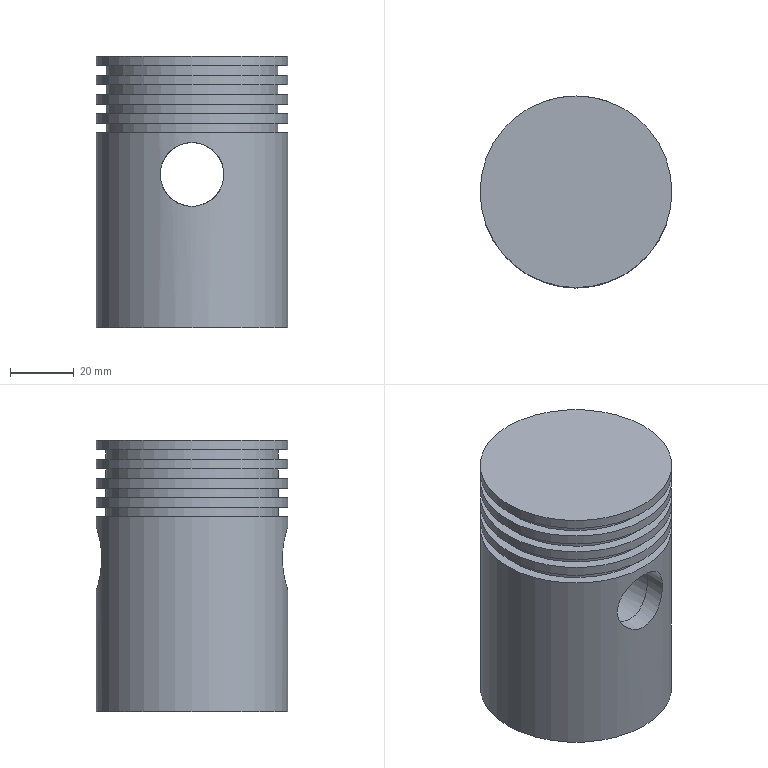Component | NX | PISTON_3 | 10 solids | 41 faces | volume 103383 mm3 | cylinder 22 | plane 19 | commonest cylinder face diameters 48 x7 60 x5 54 x4 20 x4 26 x2